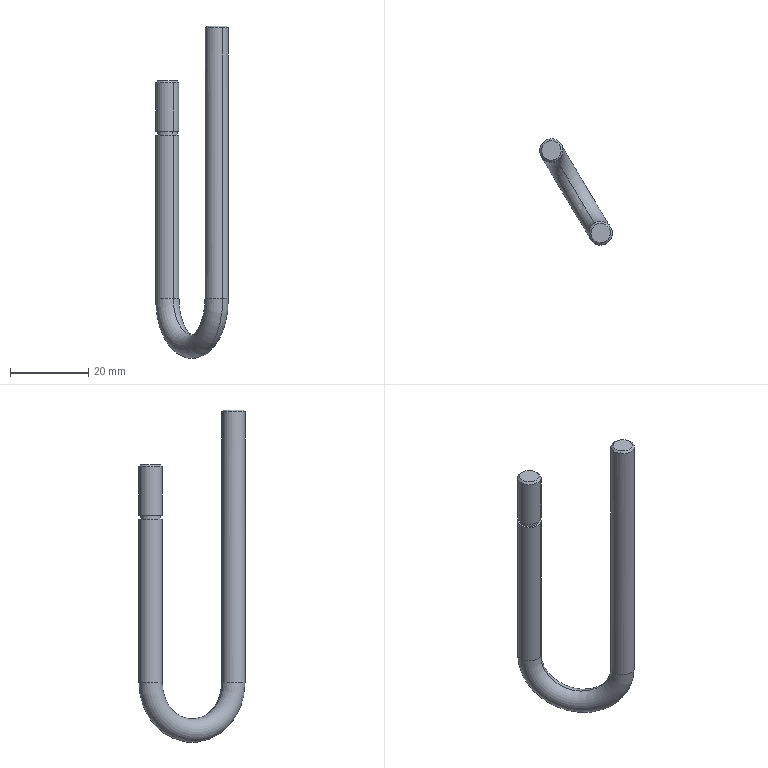Component | SolidWorks | LeftDoorAssembly-1_Bolt-1 | 1 solid | 18 faces | box 18.66 x 27.2 x 85.2 mm | volume 4638 mm3 | cylinder 8 | cone 4 | plane 4 | torus 2 | commonest cylinder face diameters 6 x6 5 x2
build123d program:
from build123d import *

# Parameters (mm, degrees)
SKETCH1_R     = 3
SKETCH3_W     = 0.5
SKETCH3_H     = 1
CHAMFER1_SIZE = 0.5


with BuildPart() as part:
    # Sweep1: sweep along a path in Sketch2
    with BuildLine(Plane.XY) as sweep1_path:
        Line((0, 0), (0, -55.85))
        ThreePointArc((0, -55.85), (12.347, -68.197), (24.694, -55.85))
        Line((24.694, -55.85), (24.694, 14))
    # Sketch1 → Sweep1 (sweep)
    with BuildSketch(Plane(origin=(0, 0, 0), x_dir=(1, 0, 0), z_dir=(0, 1, 0))):
        Circle(SKETCH1_R)
    sweep(path=sweep1_path.line)

    # Sketch3 → Cut-Revolve1 (revolve, cut)
    with BuildSketch(Plane(origin=(0, 0, 0), x_dir=(0, 0, -1), z_dir=(1, 0, 0)), mode=Mode.PRIVATE) as cut_revolve1_sk:
        with Locations((2.75, -13.5)):
            Rectangle(SKETCH3_W, SKETCH3_H)
    revolve(cut_revolve1_sk.sketch.rotate(Axis((0, 0, 0), (0, -1, 0)), 270), axis=Axis((0, 0, 0), (0, -1, 0)), mode=Mode.SUBTRACT)

    # Chamfer1
    chamfer1_edges = [part.edges().sort_by_distance(p)[0] for p in [
        (-3, 0, 0),
        (27.694, 14, 0),
    ]]
    chamfer(chamfer1_edges, length=CHAMFER1_SIZE)


solid = part.part

# Placed as in the assembly
solid = solid.moved(Location((263.17, 217.476, 1545.653), (90, -59.162, 0)))
STEP:
#1=COLOUR_RGB('',0.7922,0.8196,0.9333);
#2=FILL_AREA_STYLE_COLOUR('',#1);
#3=FILL_AREA_STYLE('',(#2));
#4=SURFACE_STYLE_FILL_AREA(#3);
#5=SURFACE_SIDE_STYLE('',(#4));
#6=SURFACE_STYLE_USAGE(.BOTH.,#5);
#7=PRESENTATION_STYLE_ASSIGNMENT((#6));
#8=CARTESIAN_POINT('',(10.3,8.663,58.654));
#9=VERTEX_POINT('',#8);
#10=CARTESIAN_POINT('',(10.422,8.461,58.654));
#11=VERTEX_POINT('',#10);
#12=CARTESIAN_POINT('',(10.361,8.562,58.654));
#13=DIRECTION('',(-0.,0.,1.));
#14=DIRECTION('',(-0.8586,-0.5126,0.));
#15=AXIS2_PLACEMENT_3D('',#12,#13,#14);
#16=CIRCLE('',#15,0.1181);
#17=EDGE_CURVE('',#9,#11,#16,.T.);
#18=ORIENTED_EDGE('',*,*,#17,.F.);
#19=CARTESIAN_POINT('',(10.92,7.626,58.654));
#20=VERTEX_POINT('',#19);
#21=CARTESIAN_POINT('',(10.61,8.145,58.654));
#22=DIRECTION('',(-0.8586,-0.5126,-0.));
#23=DIRECTION('',(0.5126,-0.8586,0.));
#24=AXIS2_PLACEMENT_3D('',#21,#22,#23);
#25=CIRCLE('',#24,0.6042);
#26=EDGE_CURVE('',#9,#20,#25,.T.);
#27=ORIENTED_EDGE('',*,*,#26,.T.);
#28=CARTESIAN_POINT('',(10.799,7.829,58.654));
#29=VERTEX_POINT('',#28);
#30=CARTESIAN_POINT('',(10.859,7.727,58.654));
#31=DIRECTION('',(0.,-0.,-1.));
#32=DIRECTION('',(-0.8586,-0.5126,0.));
#33=AXIS2_PLACEMENT_3D('',#30,#31,#32);
#34=CIRCLE('',#33,0.1181);
#35=EDGE_CURVE('',#20,#29,#34,.T.);
#36=ORIENTED_EDGE('',*,*,#35,.T.);
#37=CARTESIAN_POINT('',(10.61,8.145,58.654));
#38=DIRECTION('',(-0.8586,-0.5126,-0.));
#39=DIRECTION('',(0.5126,-0.8586,0.));
#40=AXIS2_PLACEMENT_3D('',#37,#38,#39);
#41=CIRCLE('',#40,0.368);
#42=EDGE_CURVE('',#11,#29,#41,.T.);
#43=ORIENTED_EDGE('',*,*,#42,.F.);
#44=EDGE_LOOP('',(#18,#27,#36,#43));
#45=FACE_OUTER_BOUND('',#44,.T.);
#46=CARTESIAN_POINT('',(10.61,8.145,58.654));
#47=DIRECTION('',(-0.8586,-0.5126,-0.));
#48=DIRECTION('',(0.5126,-0.8586,0.));
#49=AXIS2_PLACEMENT_3D('',#46,#47,#48);
#50=TOROIDAL_SURFACE('',#49,0.4861,0.1181);
#51=ADVANCED_FACE('',(#45),#50,.T.);
#52=CARTESIAN_POINT('',(10.775,7.677,61.404));
#53=VERTEX_POINT('',#52);
#54=CARTESIAN_POINT('',(10.944,7.778,61.404));
#55=VERTEX_POINT('',#54);
#56=CARTESIAN_POINT('',(10.859,7.727,61.404));
#57=DIRECTION('',(-0.,0.,1.));
#58=DIRECTION('',(0.5126,-0.8586,0.));
#59=AXIS2_PLACEMENT_3D('',#56,#57,#58);
#60=CIRCLE('',#59,0.09843);
#61=EDGE_CURVE('',#53,#55,#60,.T.);
#62=ORIENTED_EDGE('',*,*,#61,.F.);
#63=CARTESIAN_POINT('',(10.758,7.667,61.384));
#64=VERTEX_POINT('',#63);
#65=CARTESIAN_POINT('',(10.758,7.667,61.384));
#66=DIRECTION('',(-0.6071,-0.3625,-0.7071));
#67=VECTOR('',#66,39.37);
#68=LINE('',#65,#67);
#69=EDGE_CURVE('',#53,#64,#68,.T.);
#70=ORIENTED_EDGE('',*,*,#69,.T.);
#71=CARTESIAN_POINT('',(10.92,7.626,61.384));
#72=VERTEX_POINT('',#71);
#73=CARTESIAN_POINT('',(10.859,7.727,61.384));
#74=DIRECTION('',(0.,-0.,-1.));
#75=DIRECTION('',(0.8586,0.5126,0.));
#76=AXIS2_PLACEMENT_3D('',#73,#74,#75);
#77=CIRCLE('',#76,0.1181);
#78=EDGE_CURVE('',#72,#64,#77,.T.);
#79=ORIENTED_EDGE('',*,*,#78,.F.);
#80=CARTESIAN_POINT('',(10.961,7.788,61.384));
#81=VERTEX_POINT('',#80);
#82=CARTESIAN_POINT('',(10.859,7.727,61.384));
#83=DIRECTION('',(0.,-0.,-1.));
#84=DIRECTION('',(0.8586,0.5126,0.));
#85=AXIS2_PLACEMENT_3D('',#82,#83,#84);
#86=CIRCLE('',#85,0.1181);
#87=EDGE_CURVE('',#81,#72,#86,.T.);
#88=ORIENTED_EDGE('',*,*,#87,.F.);
#89=CARTESIAN_POINT('',(10.961,7.788,61.384));
#90=DIRECTION('',(0.6071,0.3625,-0.7071));
#91=VECTOR('',#90,39.37);
#92=LINE('',#89,#91);
#93=EDGE_CURVE('',#55,#81,#92,.T.);
#94=ORIENTED_EDGE('',*,*,#93,.F.);
#95=EDGE_LOOP('',(#62,#70,#79,#88,#94));
#96=FACE_OUTER_BOUND('',#95,.T.);
#97=CARTESIAN_POINT('',(10.859,7.727,61.384));
#98=DIRECTION('',(0.,-0.,-1.));
#99=DIRECTION('',(0.8586,0.5126,0.));
#100=AXIS2_PLACEMENT_3D('',#97,#98,#99);
#101=CONICAL_SURFACE('',#100,0.1181,0.7854);
#102=ADVANCED_FACE('',(#96),#101,.T.);
#103=CARTESIAN_POINT('',(10.311,8.647,60.852));
#104=VERTEX_POINT('',#103);
#105=CARTESIAN_POINT('',(10.411,8.478,60.852));
#106=VERTEX_POINT('',#105);
#107=CARTESIAN_POINT('',(10.361,8.562,60.852));
#108=DIRECTION('',(-0.,0.,1.));
#109=DIRECTION('',(-0.8586,-0.5126,0.));
#110=AXIS2_PLACEMENT_3D('',#107,#108,#109);
#111=CIRCLE('',#110,0.09843);
#112=EDGE_CURVE('',#104,#106,#111,.T.);
#113=ORIENTED_EDGE('',*,*,#112,.F.);
#114=CARTESIAN_POINT('',(10.3,8.663,60.833));
#115=VERTEX_POINT('',#114);
#116=CARTESIAN_POINT('',(10.311,8.647,60.852));
#117=DIRECTION('',(-0.3625,0.6071,-0.7071));
#118=VECTOR('',#117,39.37);
#119=LINE('',#116,#118);
#120=EDGE_CURVE('',#104,#115,#119,.T.);
#121=ORIENTED_EDGE('',*,*,#120,.T.);
#122=CARTESIAN_POINT('',(10.422,8.461,60.833));
#123=VERTEX_POINT('',#122);
#124=CARTESIAN_POINT('',(10.361,8.562,60.833));
#125=DIRECTION('',(0.,-0.,-1.));
#126=DIRECTION('',(-0.5126,0.8586,0.));
#127=AXIS2_PLACEMENT_3D('',#124,#125,#126);
#128=CIRCLE('',#127,0.1181);
#129=EDGE_CURVE('',#123,#115,#128,.T.);
#130=ORIENTED_EDGE('',*,*,#129,.F.);
#131=CARTESIAN_POINT('',(10.411,8.478,60.852));
#132=DIRECTION('',(0.3625,-0.6071,-0.7071));
#133=VECTOR('',#132,39.37);
#134=LINE('',#131,#133);
#135=EDGE_CURVE('',#106,#123,#134,.T.);
#136=ORIENTED_EDGE('',*,*,#135,.F.);
#137=EDGE_LOOP('',(#113,#121,#130,#136));
#138=FACE_OUTER_BOUND('',#137,.T.);
#139=CARTESIAN_POINT('',(10.361,8.562,60.852));
#140=DIRECTION('',(0.,-0.,-1.));
#141=DIRECTION('',(0.5126,-0.8586,0.));
#142=AXIS2_PLACEMENT_3D('',#139,#140,#141);
#143=CONICAL_SURFACE('',#142,0.09843,0.7854);
#144=ADVANCED_FACE('',(#138),#143,.T.);
#145=CARTESIAN_POINT('',(10.3,8.663,60.341));
#146=VERTEX_POINT('',#145);
#147=CARTESIAN_POINT('',(10.422,8.461,60.341));
#148=VERTEX_POINT('',#147);
#149=CARTESIAN_POINT('',(10.361,8.562,60.341));
#150=DIRECTION('',(-0.,0.,1.));
#151=DIRECTION('',(-0.5126,0.8586,0.));
#152=AXIS2_PLACEMENT_3D('',#149,#150,#151);
#153=CIRCLE('',#152,0.1181);
#154=EDGE_CURVE('',#146,#148,#153,.T.);
#155=ORIENTED_EDGE('',*,*,#154,.T.);
#156=CARTESIAN_POINT('',(10.422,8.461,58.654));
#157=DIRECTION('',(-0.,0.,1.));
#158=VECTOR('',#157,39.37);
#159=LINE('',#156,#158);
#160=EDGE_CURVE('',#148,#123,#159,.T.);
#161=ORIENTED_EDGE('',*,*,#160,.T.);
#162=ORIENTED_EDGE('',*,*,#129,.T.);
#163=CARTESIAN_POINT('',(10.3,8.663,58.654));
#164=DIRECTION('',(-0.,0.,1.));
#165=VECTOR('',#164,39.37);
#166=LINE('',#163,#165);
#167=EDGE_CURVE('',#146,#115,#166,.T.);
#168=ORIENTED_EDGE('',*,*,#167,.F.);
#169=EDGE_LOOP('',(#155,#161,#162,#168));
#170=FACE_OUTER_BOUND('',#169,.T.);
#171=CARTESIAN_POINT('',(10.361,8.562,58.654));
#172=DIRECTION('',(-0.,0.,1.));
#173=DIRECTION('',(-0.5126,0.8586,0.));
#174=AXIS2_PLACEMENT_3D('',#171,#172,#173);
#175=CYLINDRICAL_SURFACE('',#174,0.1181);
#176=ADVANCED_FACE('',(#170),#175,.T.);
#177=CARTESIAN_POINT('',(10.311,8.647,60.301));
#178=VERTEX_POINT('',#177);
#179=CARTESIAN_POINT('',(10.411,8.478,60.301));
#180=VERTEX_POINT('',#179);
#181=CARTESIAN_POINT('',(10.361,8.562,60.301));
#182=DIRECTION('',(-0.,0.,1.));
#183=DIRECTION('',(-0.5126,0.8586,0.));
#184=AXIS2_PLACEMENT_3D('',#181,#182,#183);
#185=CIRCLE('',#184,0.09843);
#186=EDGE_CURVE('',#178,#180,#185,.T.);
#187=ORIENTED_EDGE('',*,*,#186,.T.);
#188=CARTESIAN_POINT('',(10.411,8.478,60.341));
#189=VERTEX_POINT('',#188);
#190=CARTESIAN_POINT('',(10.411,8.478,60.852));
#191=DIRECTION('',(-0.,0.,1.));
#192=VECTOR('',#191,39.37);
#193=LINE('',#190,#192);
#194=EDGE_CURVE('',#180,#189,#193,.T.);
#195=ORIENTED_EDGE('',*,*,#194,.T.);
#196=CARTESIAN_POINT('',(10.311,8.647,60.341));
#197=VERTEX_POINT('',#196);
#198=CARTESIAN_POINT('',(10.361,8.562,60.341));
#199=DIRECTION('',(-0.,0.,1.));
#200=DIRECTION('',(-0.5126,0.8586,0.));
#201=AXIS2_PLACEMENT_3D('',#198,#199,#200);
#202=CIRCLE('',#201,0.09843);
#203=EDGE_CURVE('',#197,#189,#202,.T.);
#204=ORIENTED_EDGE('',*,*,#203,.F.);
#205=CARTESIAN_POINT('',(10.311,8.647,60.852));
#206=DIRECTION('',(-0.,0.,1.));
#207=VECTOR('',#206,39.37);
#208=LINE('',#205,#207);
#209=EDGE_CURVE('',#178,#197,#208,.T.);
#210=ORIENTED_EDGE('',*,*,#209,.F.);
#211=EDGE_LOOP('',(#187,#195,#204,#210));
#212=FACE_OUTER_BOUND('',#211,.T.);
#213=CARTESIAN_POINT('',(10.361,8.562,60.852));
#214=DIRECTION('',(-0.,0.,1.));
#215=DIRECTION('',(-0.5126,0.8586,0.));
#216=AXIS2_PLACEMENT_3D('',#213,#214,#215);
#217=CYLINDRICAL_SURFACE('',#216,0.09843);
#218=ADVANCED_FACE('',(#212),#217,.T.);
#219=ORIENTED_EDGE('',*,*,#35,.F.);
#220=CARTESIAN_POINT('',(10.92,7.626,58.654));
#221=DIRECTION('',(-0.,0.,1.));
#222=VECTOR('',#221,39.37);
#223=LINE('',#220,#222);
#224=EDGE_CURVE('',#20,#72,#223,.T.);
#225=ORIENTED_EDGE('',*,*,#224,.T.);
#226=ORIENTED_EDGE('',*,*,#78,.T.);
#227=CARTESIAN_POINT('',(10.799,7.829,61.384));
#228=VERTEX_POINT('',#227);
#229=CARTESIAN_POINT('',(10.859,7.727,61.384));
#230=DIRECTION('',(0.,-0.,-1.));
#231=DIRECTION('',(0.8586,0.5126,0.));
#232=AXIS2_PLACEMENT_3D('',#229,#230,#231);
#233=CIRCLE('',#232,0.1181);
#234=EDGE_CURVE('',#64,#228,#233,.T.);
#235=ORIENTED_EDGE('',*,*,#234,.T.);
#236=CARTESIAN_POINT('',(10.799,7.829,58.654));
#237=DIRECTION('',(-0.,0.,1.));
#238=VECTOR('',#237,39.37);
#239=LINE('',#236,#238);
#240=EDGE_CURVE('',#29,#228,#239,.T.);
#241=ORIENTED_EDGE('',*,*,#240,.F.);
#242=EDGE_LOOP('',(#219,#225,#226,#235,#241));
#243=FACE_OUTER_BOUND('',#242,.T.);
#244=CARTESIAN_POINT('',(10.859,7.727,58.654));
#245=DIRECTION('',(-0.,0.,1.));
#246=DIRECTION('',(-0.5126,0.8586,0.));
#247=AXIS2_PLACEMENT_3D('',#244,#245,#246);
#248=CYLINDRICAL_SURFACE('',#247,0.1181);
#249=ADVANCED_FACE('',(#243),#248,.T.);
#250=ORIENTED_EDGE('',*,*,#17,.T.);
#251=CARTESIAN_POINT('',(10.422,8.461,60.301));
#252=VERTEX_POINT('',#251);
#253=CARTESIAN_POINT('',(10.422,8.461,58.654));
#254=DIRECTION('',(-0.,0.,1.));
#255=VECTOR('',#254,39.37);
#256=LINE('',#253,#255);
#257=EDGE_CURVE('',#11,#252,#256,.T.);
#258=ORIENTED_EDGE('',*,*,#257,.T.);
#259=CARTESIAN_POINT('',(10.3,8.663,60.301));
#260=VERTEX_POINT('',#259);
#261=CARTESIAN_POINT('',(10.361,8.562,60.301));
#262=DIRECTION('',(-0.,0.,1.));
#263=DIRECTION('',(-0.5126,0.8586,0.));
#264=AXIS2_PLACEMENT_3D('',#261,#262,#263);
#265=CIRCLE('',#264,0.1181);
#266=EDGE_CURVE('',#260,#252,#265,.T.);
#267=ORIENTED_EDGE('',*,*,#266,.F.);
#268=CARTESIAN_POINT('',(10.3,8.663,58.654));
#269=DIRECTION('',(-0.,0.,1.));
#270=VECTOR('',#269,39.37);
#271=LINE('',#268,#270);
#272=EDGE_CURVE('',#9,#260,#271,.T.);
#273=ORIENTED_EDGE('',*,*,#272,.F.);
#274=EDGE_LOOP('',(#250,#258,#267,#273));
#275=FACE_OUTER_BOUND('',#274,.T.);
#276=CARTESIAN_POINT('',(10.361,8.562,58.654));
#277=DIRECTION('',(-0.,0.,1.));
#278=DIRECTION('',(-0.5126,0.8586,0.));
#279=AXIS2_PLACEMENT_3D('',#276,#277,#278);
#280=CYLINDRICAL_SURFACE('',#279,0.1181);
#281=ADVANCED_FACE('',(#275),#280,.T.);
#282=ORIENTED_EDGE('',*,*,#257,.F.);
#283=CARTESIAN_POINT('',(10.361,8.562,58.654));
#284=DIRECTION('',(-0.,0.,1.));
#285=DIRECTION('',(-0.8586,-0.5126,0.));
#286=AXIS2_PLACEMENT_3D('',#283,#284,#285);
#287=CIRCLE('',#286,0.1181);
#288=EDGE_CURVE('',#11,#9,#287,.T.);
#289=ORIENTED_EDGE('',*,*,#288,.T.);
#290=ORIENTED_EDGE('',*,*,#272,.T.);
#291=CARTESIAN_POINT('',(10.361,8.562,60.301));
#292=DIRECTION('',(-0.,0.,1.));
#293=DIRECTION('',(-0.5126,0.8586,0.));
#294=AXIS2_PLACEMENT_3D('',#291,#292,#293);
#295=CIRCLE('',#294,0.1181);
#296=EDGE_CURVE('',#252,#260,#295,.T.);
#297=ORIENTED_EDGE('',*,*,#296,.F.);
#298=EDGE_LOOP('',(#282,#289,#290,#297));
#299=FACE_OUTER_BOUND('',#298,.T.);
#300=CARTESIAN_POINT('',(10.361,8.562,58.654));
#301=DIRECTION('',(-0.,0.,1.));
#302=DIRECTION('',(-0.5126,0.8586,0.));
#303=AXIS2_PLACEMENT_3D('',#300,#301,#302);
#304=CYLINDRICAL_SURFACE('',#303,0.1181);
#305=ADVANCED_FACE('',(#299),#304,.T.);
#306=ORIENTED_EDGE('',*,*,#224,.F.);
#307=CARTESIAN_POINT('',(10.859,7.727,58.654));
#308=DIRECTION('',(0.,-0.,-1.));
#309=DIRECTION('',(-0.8586,-0.5126,0.));
#310=AXIS2_PLACEMENT_3D('',#307,#308,#309);
#311=CIRCLE('',#310,0.1181);
#312=EDGE_CURVE('',#29,#20,#311,.T.);
#313=ORIENTED_EDGE('',*,*,#312,.F.);
#314=ORIENTED_EDGE('',*,*,#240,.T.);
#315=CARTESIAN_POINT('',(10.859,7.727,61.384));
#316=DIRECTION('',(0.,-0.,-1.));
#317=DIRECTION('',(0.8586,0.5126,0.));
#318=AXIS2_PLACEMENT_3D('',#315,#316,#317);
#319=CIRCLE('',#318,0.1181);
#320=EDGE_CURVE('',#228,#81,#319,.T.);
#321=ORIENTED_EDGE('',*,*,#320,.T.);
#322=ORIENTED_EDGE('',*,*,#87,.T.);
#323=EDGE_LOOP('',(#306,#313,#314,#321,#322));
#324=FACE_OUTER_BOUND('',#323,.T.);
#325=CARTESIAN_POINT('',(10.859,7.727,58.654));
#326=DIRECTION('',(-0.,0.,1.));
#327=DIRECTION('',(-0.5126,0.8586,0.));
#328=AXIS2_PLACEMENT_3D('',#325,#326,#327);
#329=CYLINDRICAL_SURFACE('',#328,0.1181);
#330=ADVANCED_FACE('',(#324),#329,.T.);
#331=ORIENTED_EDGE('',*,*,#26,.F.);
#332=ORIENTED_EDGE('',*,*,#288,.F.);
#333=ORIENTED_EDGE('',*,*,#42,.T.);
#334=ORIENTED_EDGE('',*,*,#312,.T.);
#335=EDGE_LOOP('',(#331,#332,#333,#334));
#336=FACE_OUTER_BOUND('',#335,.T.);
#337=CARTESIAN_POINT('',(10.61,8.145,58.654));
#338=DIRECTION('',(-0.8586,-0.5126,-0.));
#339=DIRECTION('',(0.5126,-0.8586,0.));
#340=AXIS2_PLACEMENT_3D('',#337,#338,#339);
#341=TOROIDAL_SURFACE('',#340,0.4861,0.1181);
#342=ADVANCED_FACE('',(#336),#341,.T.);
#343=CARTESIAN_POINT('',(10.859,7.727,61.404));
#344=DIRECTION('',(-0.,0.,1.));
#345=DIRECTION('',(0.5126,-0.8586,0.));
#346=AXIS2_PLACEMENT_3D('',#343,#344,#345);
#347=CIRCLE('',#346,0.09843);
#348=EDGE_CURVE('',#55,#53,#347,.T.);
#349=ORIENTED_EDGE('',*,*,#348,.T.);
#350=ORIENTED_EDGE('',*,*,#61,.T.);
#351=EDGE_LOOP('',(#349,#350));
#352=FACE_OUTER_BOUND('',#351,.T.);
#353=CARTESIAN_POINT('',(10.859,7.727,61.404));
#354=DIRECTION('',(0.,-0.,-1.));
#355=DIRECTION('',(-0.8586,-0.5126,-0.));
#356=AXIS2_PLACEMENT_3D('',#353,#354,#355);
#357=PLANE('',#356);
#358=ADVANCED_FACE('',(#352),#357,.F.);
#359=ORIENTED_EDGE('',*,*,#194,.F.);
#360=CARTESIAN_POINT('',(10.361,8.562,60.301));
#361=DIRECTION('',(-0.,0.,1.));
#362=DIRECTION('',(-0.5126,0.8586,0.));
#363=AXIS2_PLACEMENT_3D('',#360,#361,#362);
#364=CIRCLE('',#363,0.09843);
#365=EDGE_CURVE('',#180,#178,#364,.T.);
#366=ORIENTED_EDGE('',*,*,#365,.T.);
#367=ORIENTED_EDGE('',*,*,#209,.T.);
#368=CARTESIAN_POINT('',(10.361,8.562,60.341));
#369=DIRECTION('',(-0.,0.,1.));
#370=DIRECTION('',(-0.5126,0.8586,0.));
#371=AXIS2_PLACEMENT_3D('',#368,#369,#370);
#372=CIRCLE('',#371,0.09843);
#373=EDGE_CURVE('',#189,#197,#372,.T.);
#374=ORIENTED_EDGE('',*,*,#373,.F.);
#375=EDGE_LOOP('',(#359,#366,#367,#374));
#376=FACE_OUTER_BOUND('',#375,.T.);
#377=CARTESIAN_POINT('',(10.361,8.562,60.852));
#378=DIRECTION('',(-0.,0.,1.));
#379=DIRECTION('',(-0.5126,0.8586,0.));
#380=AXIS2_PLACEMENT_3D('',#377,#378,#379);
#381=CYLINDRICAL_SURFACE('',#380,0.09843);
#382=ADVANCED_FACE('',(#376),#381,.T.);
#383=ORIENTED_EDGE('',*,*,#203,.T.);
#384=ORIENTED_EDGE('',*,*,#373,.T.);
#385=EDGE_LOOP('',(#383,#384));
#386=FACE_BOUND('',#385,.T.);
#387=ORIENTED_EDGE('',*,*,#154,.F.);
#388=CARTESIAN_POINT('',(10.361,8.562,60.341));
#389=DIRECTION('',(-0.,0.,1.));
#390=DIRECTION('',(-0.5126,0.8586,0.));
#391=AXIS2_PLACEMENT_3D('',#388,#389,#390);
#392=CIRCLE('',#391,0.1181);
#393=EDGE_CURVE('',#148,#146,#392,.T.);
#394=ORIENTED_EDGE('',*,*,#393,.F.);
#395=EDGE_LOOP('',(#387,#394));
#396=FACE_OUTER_BOUND('',#395,.T.);
#397=CARTESIAN_POINT('',(10.446,8.613,60.341));
#398=DIRECTION('',(0.,-0.,-1.));
#399=DIRECTION('',(0.5126,-0.8586,0.));
#400=AXIS2_PLACEMENT_3D('',#397,#398,#399);
#401=PLANE('',#400);
#402=ADVANCED_FACE('',(#386,#396),#401,.T.);
#403=ORIENTED_EDGE('',*,*,#266,.T.);
#404=ORIENTED_EDGE('',*,*,#296,.T.);
#405=EDGE_LOOP('',(#403,#404));
#406=FACE_OUTER_BOUND('',#405,.T.);
#407=ORIENTED_EDGE('',*,*,#186,.F.);
#408=ORIENTED_EDGE('',*,*,#365,.F.);
#409=EDGE_LOOP('',(#407,#408));
#410=FACE_BOUND('',#409,.T.);
#411=CARTESIAN_POINT('',(10.446,8.613,60.301));
#412=DIRECTION('',(-0.,0.,1.));
#413=DIRECTION('',(-0.5126,0.8586,-0.));
#414=AXIS2_PLACEMENT_3D('',#411,#412,#413);
#415=PLANE('',#414);
#416=ADVANCED_FACE('',(#406,#410),#415,.T.);
#417=CARTESIAN_POINT('',(10.361,8.562,60.852));
#418=DIRECTION('',(-0.,0.,1.));
#419=DIRECTION('',(-0.8586,-0.5126,0.));
#420=AXIS2_PLACEMENT_3D('',#417,#418,#419);
#421=CIRCLE('',#420,0.09843);
#422=EDGE_CURVE('',#106,#104,#421,.T.);
#423=ORIENTED_EDGE('',*,*,#422,.T.);
#424=ORIENTED_EDGE('',*,*,#112,.T.);
#425=EDGE_LOOP('',(#423,#424));
#426=FACE_OUTER_BOUND('',#425,.T.);
#427=CARTESIAN_POINT('',(10.361,8.562,60.852));
#428=DIRECTION('',(-0.,0.,1.));
#429=DIRECTION('',(-0.8586,-0.5126,-0.));
#430=AXIS2_PLACEMENT_3D('',#427,#428,#429);
#431=PLANE('',#430);
#432=ADVANCED_FACE('',(#426),#431,.T.);
#433=ORIENTED_EDGE('',*,*,#160,.F.);
#434=ORIENTED_EDGE('',*,*,#393,.T.);
#435=ORIENTED_EDGE('',*,*,#167,.T.);
#436=CARTESIAN_POINT('',(10.361,8.562,60.833));
#437=DIRECTION('',(0.,-0.,-1.));
#438=DIRECTION('',(-0.5126,0.8586,0.));
#439=AXIS2_PLACEMENT_3D('',#436,#437,#438);
#440=CIRCLE('',#439,0.1181);
#441=EDGE_CURVE('',#115,#123,#440,.T.);
#442=ORIENTED_EDGE('',*,*,#441,.T.);
#443=EDGE_LOOP('',(#433,#434,#435,#442));
#444=FACE_OUTER_BOUND('',#443,.T.);
#445=CARTESIAN_POINT('',(10.361,8.562,58.654));
#446=DIRECTION('',(-0.,0.,1.));
#447=DIRECTION('',(-0.5126,0.8586,0.));
#448=AXIS2_PLACEMENT_3D('',#445,#446,#447);
#449=CYLINDRICAL_SURFACE('',#448,0.1181);
#450=ADVANCED_FACE('',(#444),#449,.T.);
#451=ORIENTED_EDGE('',*,*,#120,.F.);
#452=ORIENTED_EDGE('',*,*,#422,.F.);
#453=ORIENTED_EDGE('',*,*,#135,.T.);
#454=ORIENTED_EDGE('',*,*,#441,.F.);
#455=EDGE_LOOP('',(#451,#452,#453,#454));
#456=FACE_OUTER_BOUND('',#455,.T.);
#457=CARTESIAN_POINT('',(10.361,8.562,60.852));
#458=DIRECTION('',(0.,-0.,-1.));
#459=DIRECTION('',(0.5126,-0.8586,0.));
#460=AXIS2_PLACEMENT_3D('',#457,#458,#459);
#461=CONICAL_SURFACE('',#460,0.09843,0.7854);
#462=ADVANCED_FACE('',(#456),#461,.T.);
#463=ORIENTED_EDGE('',*,*,#69,.F.);
#464=ORIENTED_EDGE('',*,*,#348,.F.);
#465=ORIENTED_EDGE('',*,*,#93,.T.);
#466=ORIENTED_EDGE('',*,*,#320,.F.);
#467=ORIENTED_EDGE('',*,*,#234,.F.);
#468=EDGE_LOOP('',(#463,#464,#465,#466,#467));
#469=FACE_OUTER_BOUND('',#468,.T.);
#470=CARTESIAN_POINT('',(10.859,7.727,61.384));
#471=DIRECTION('',(0.,-0.,-1.));
#472=DIRECTION('',(0.8586,0.5126,0.));
#473=AXIS2_PLACEMENT_3D('',#470,#471,#472);
#474=CONICAL_SURFACE('',#473,0.1181,0.7854);
#475=ADVANCED_FACE('',(#469),#474,.T.);
#476=CLOSED_SHELL('',(#51,#102,#144,#176,#218,#249,#281,#305,#330,#342,#358,#382,#402,#416,#432,#450,#462,#475));
#477=MANIFOLD_SOLID_BREP('',#476);
#478=STYLED_ITEM('',(#7),#477);
#479=PRESENTATION_LAYER_ASSIGNMENT('','',(#478));
#480=(LENGTH_UNIT()NAMED_UNIT(*)SI_UNIT($,.METRE.));
#481=LENGTH_MEASURE_WITH_UNIT(LENGTH_MEASURE(0.0254),#480);
#482=DIMENSIONAL_EXPONENTS(1.,0.,0.,0.,0.,0.,0.);
#483=(CONVERSION_BASED_UNIT('',#481)LENGTH_UNIT()NAMED_UNIT(#482));
#484=UNCERTAINTY_MEASURE_WITH_UNIT(LENGTH_MEASURE(0.00001),#483,'','');
#485=(NAMED_UNIT(*)PLANE_ANGLE_UNIT()SI_UNIT($,.RADIAN.));
#486=(NAMED_UNIT(*)SI_UNIT($,.STERADIAN.)SOLID_ANGLE_UNIT());
#487=(GEOMETRIC_REPRESENTATION_CONTEXT(3)GLOBAL_UNCERTAINTY_ASSIGNED_CONTEXT((#484))GLOBAL_UNIT_ASSIGNED_CONTEXT((#483,#485,#486))REPRESENTATION_CONTEXT('',''));
#488=MECHANICAL_DESIGN_GEOMETRIC_PRESENTATION_REPRESENTATION('',(#478),#487);
#489=CARTESIAN_POINT('',(0.,0.,0.));
#490=DIRECTION('',(0.,0.,1.));
#491=DIRECTION('',(1.,0.,0.));
#492=AXIS2_PLACEMENT_3D('',#489,#490,#491);
#493=(LENGTH_UNIT()NAMED_UNIT(*)SI_UNIT($,.METRE.));
#494=LENGTH_MEASURE_WITH_UNIT(LENGTH_MEASURE(0.0254),#493);
#495=DIMENSIONAL_EXPONENTS(1.,0.,0.,0.,0.,0.,0.);
#496=(CONVERSION_BASED_UNIT('',#494)LENGTH_UNIT()NAMED_UNIT(#495));
#497=UNCERTAINTY_MEASURE_WITH_UNIT(LENGTH_MEASURE(0.00001),#496,'','');
#498=(NAMED_UNIT(*)PLANE_ANGLE_UNIT()SI_UNIT($,.RADIAN.));
#499=(NAMED_UNIT(*)SI_UNIT($,.STERADIAN.)SOLID_ANGLE_UNIT());
#500=(GEOMETRIC_REPRESENTATION_CONTEXT(3)GLOBAL_UNCERTAINTY_ASSIGNED_CONTEXT((#497))GLOBAL_UNIT_ASSIGNED_CONTEXT((#496,#498,#499))REPRESENTATION_CONTEXT('',''));
#501=ADVANCED_BREP_SHAPE_REPRESENTATION('',(#477,#492),#500);